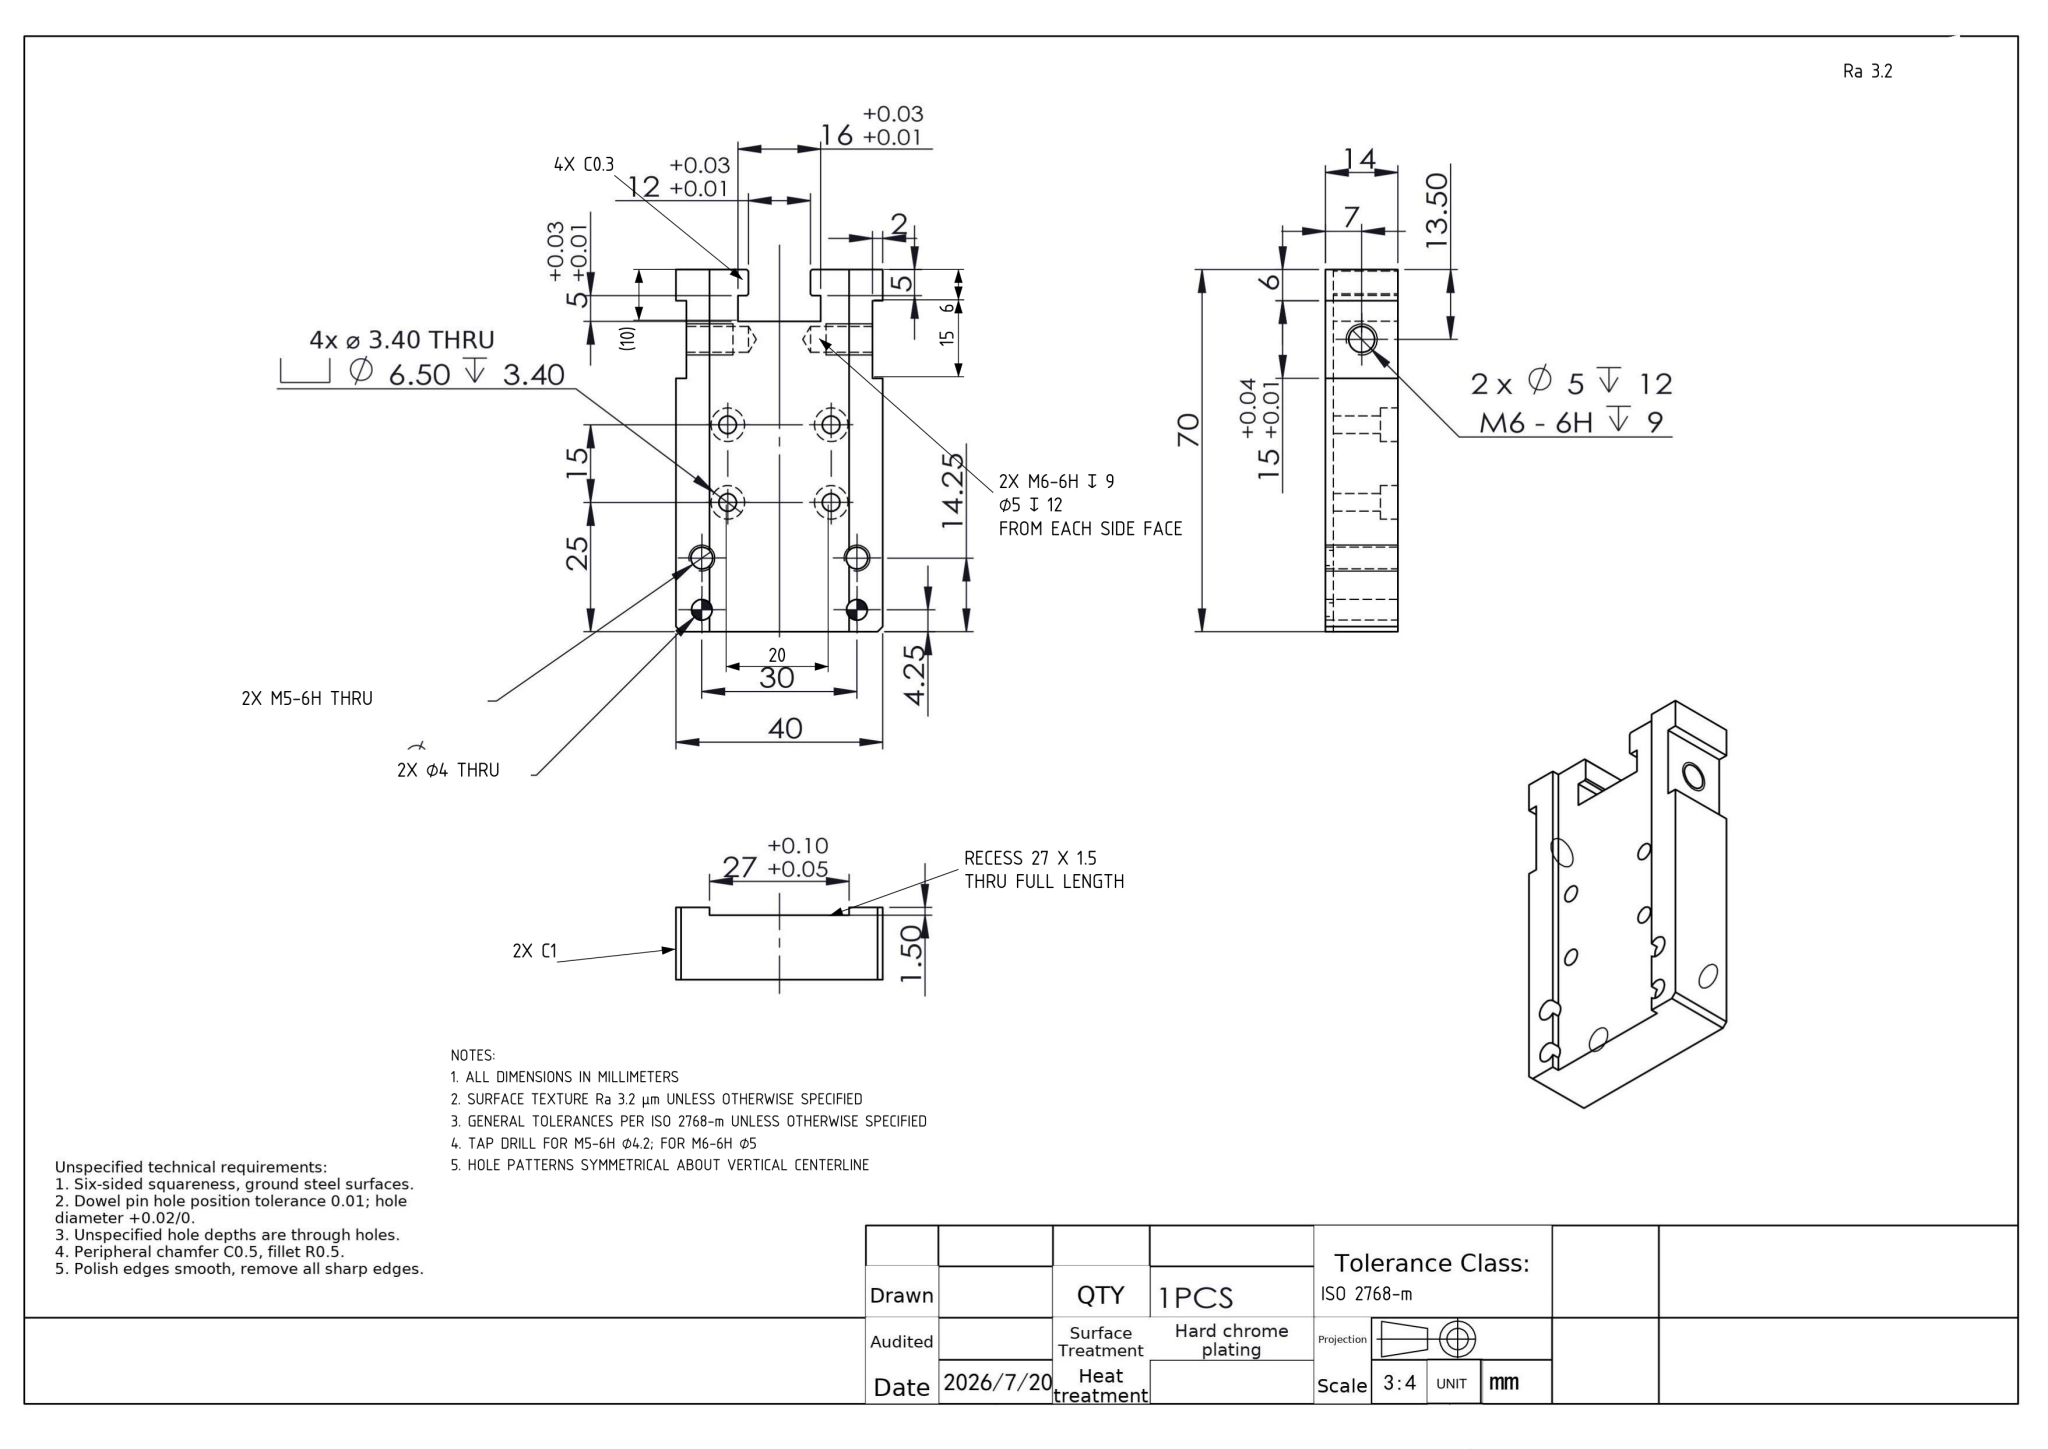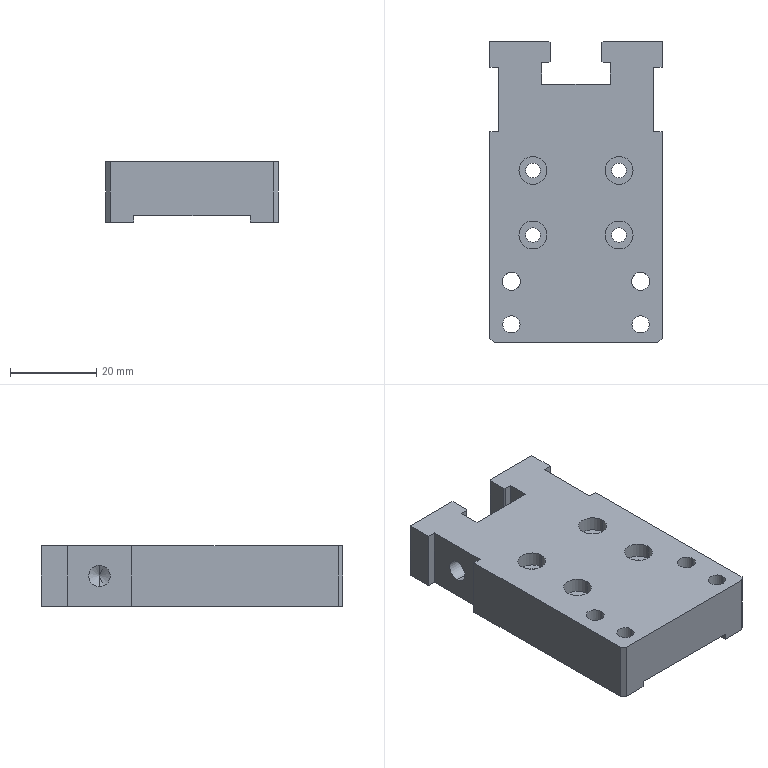Part | NX | mm | Tabbed Multi-Bore Manifold Block | 1 solid | 72 faces | box 40 x 70 x 14 mm | volume 31753 mm3 | plane 40 | cylinder 28 | cone 4 | commonest cylinder face diameters 6.5 x8 3.4 x8 4 x4 4.2 x4 5 x4